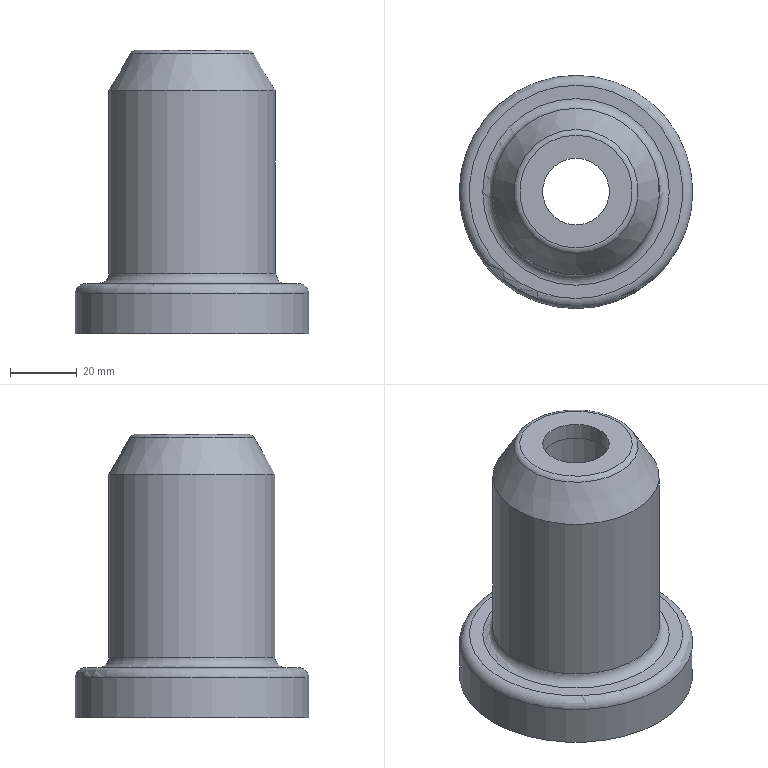Component | NX | CYLINDER | 1 solid | 32 faces | volume 103061 mm3 | cylinder 13 | cone 8 | plane 6 | torus 5 | commonest cylinder face diameters 6 x6 70 x1 50 x1 20 x1 28 x1 40 x1 46 x1 3 x1